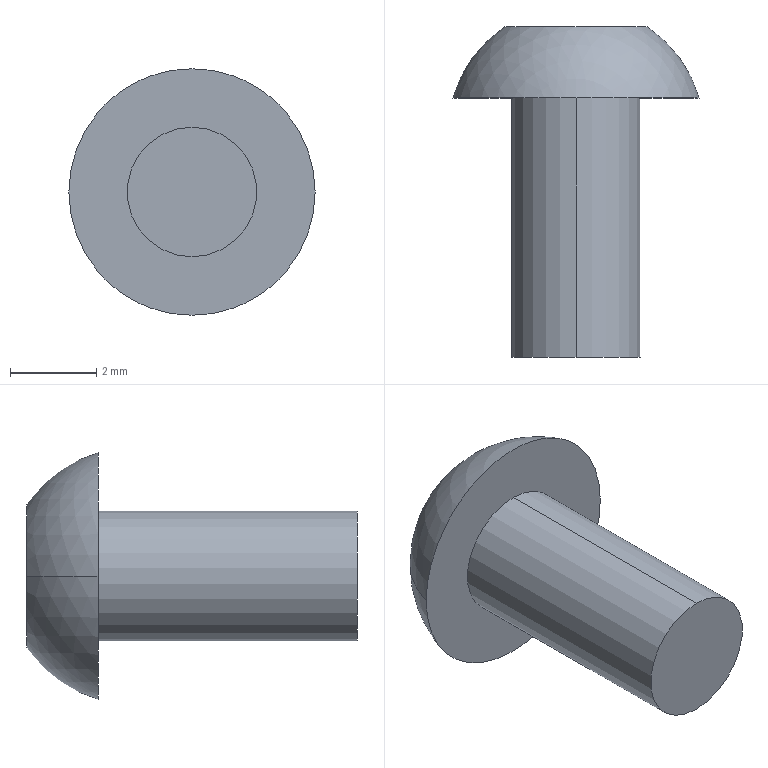Component | SolidWorks | hexagon socket button head screws gb-1 | 1 solid | 19 faces | box 5.7 x 7.65 x 5.7 mm | volume 69 mm3 | plane 15 | sphere 2 | cylinder 2 | commonest cylinder face diameters 3 x2
STEP:
#1=COLOUR_RGB('',0.7922,0.8196,0.9333);
#2=FILL_AREA_STYLE_COLOUR('',#1);
#3=FILL_AREA_STYLE('',(#2));
#4=SURFACE_STYLE_FILL_AREA(#3);
#5=SURFACE_SIDE_STYLE('',(#4));
#6=SURFACE_STYLE_USAGE(.BOTH.,#5);
#7=PRESENTATION_STYLE_ASSIGNMENT((#6));
#8=CARTESIAN_POINT('',(0.7107,0.6105,5.318));
#9=VERTEX_POINT('',#8);
#10=CARTESIAN_POINT('',(0.4863,0.6105,5.318));
#11=VERTEX_POINT('',#10);
#12=CARTESIAN_POINT('',(0.5985,0.6105,5.318));
#13=DIRECTION('',(0.,1.,-0.));
#14=DIRECTION('',(0.,0.,1.));
#15=AXIS2_PLACEMENT_3D('',#12,#13,#14);
#16=CIRCLE('',#15,0.1122);
#17=EDGE_CURVE('',#9,#11,#16,.T.);
#18=ORIENTED_EDGE('',*,*,#17,.T.);
#19=CARTESIAN_POINT('',(0.5336,0.6754,5.318));
#20=VERTEX_POINT('',#19);
#21=CARTESIAN_POINT('',(0.5985,0.5785,5.318));
#22=DIRECTION('',(0.,-0.,-1.));
#23=DIRECTION('',(-1.,0.,0.));
#24=AXIS2_PLACEMENT_3D('',#21,#22,#23);
#25=CIRCLE('',#24,0.1167);
#26=EDGE_CURVE('',#11,#20,#25,.T.);
#27=ORIENTED_EDGE('',*,*,#26,.T.);
#28=CARTESIAN_POINT('',(0.6635,0.6754,5.318));
#29=VERTEX_POINT('',#28);
#30=CARTESIAN_POINT('',(0.5985,0.6754,5.318));
#31=DIRECTION('',(0.,1.,-0.));
#32=DIRECTION('',(0.,0.,1.));
#33=AXIS2_PLACEMENT_3D('',#30,#31,#32);
#34=CIRCLE('',#33,0.06496);
#35=EDGE_CURVE('',#29,#20,#34,.T.);
#36=ORIENTED_EDGE('',*,*,#35,.F.);
#37=CARTESIAN_POINT('',(0.5985,0.5785,5.318));
#38=DIRECTION('',(-0.,0.,1.));
#39=DIRECTION('',(1.,0.,0.));
#40=AXIS2_PLACEMENT_3D('',#37,#38,#39);
#41=CIRCLE('',#40,0.1167);
#42=EDGE_CURVE('',#9,#29,#41,.T.);
#43=ORIENTED_EDGE('',*,*,#42,.F.);
#44=EDGE_LOOP('',(#18,#27,#36,#43));
#45=FACE_OUTER_BOUND('',#44,.T.);
#46=CARTESIAN_POINT('',(0.5985,0.5785,5.318));
#47=DIRECTION('',(0.,-0.,-1.));
#48=DIRECTION('',(1.,0.,0.));
#49=AXIS2_PLACEMENT_3D('',#46,#47,#48);
#50=SPHERICAL_SURFACE('',#49,0.1167);
#51=ADVANCED_FACE('',(#45),#50,.T.);
#52=CARTESIAN_POINT('',(0.5985,0.3743,5.259));
#53=VERTEX_POINT('',#52);
#54=CARTESIAN_POINT('',(0.5985,0.3743,5.377));
#55=VERTEX_POINT('',#54);
#56=CARTESIAN_POINT('',(0.5985,0.3743,5.318));
#57=DIRECTION('',(-0.,-1.,0.));
#58=DIRECTION('',(0.,0.,-1.));
#59=AXIS2_PLACEMENT_3D('',#56,#57,#58);
#60=CIRCLE('',#59,0.05906);
#61=EDGE_CURVE('',#53,#55,#60,.T.);
#62=ORIENTED_EDGE('',*,*,#61,.F.);
#63=CARTESIAN_POINT('',(0.5985,0.6105,5.259));
#64=VERTEX_POINT('',#63);
#65=CARTESIAN_POINT('',(0.5985,0.3743,5.259));
#66=DIRECTION('',(0.,1.,-0.));
#67=VECTOR('',#66,39.37);
#68=LINE('',#65,#67);
#69=EDGE_CURVE('',#53,#64,#68,.T.);
#70=ORIENTED_EDGE('',*,*,#69,.T.);
#71=CARTESIAN_POINT('',(0.5985,0.6105,5.377));
#72=VERTEX_POINT('',#71);
#73=CARTESIAN_POINT('',(0.5985,0.6105,5.318));
#74=DIRECTION('',(-0.,-1.,0.));
#75=DIRECTION('',(0.,0.,-1.));
#76=AXIS2_PLACEMENT_3D('',#73,#74,#75);
#77=CIRCLE('',#76,0.05906);
#78=EDGE_CURVE('',#64,#72,#77,.T.);
#79=ORIENTED_EDGE('',*,*,#78,.T.);
#80=CARTESIAN_POINT('',(0.5985,0.3743,5.377));
#81=DIRECTION('',(0.,1.,-0.));
#82=VECTOR('',#81,39.37);
#83=LINE('',#80,#82);
#84=EDGE_CURVE('',#55,#72,#83,.T.);
#85=ORIENTED_EDGE('',*,*,#84,.F.);
#86=EDGE_LOOP('',(#62,#70,#79,#85));
#87=FACE_OUTER_BOUND('',#86,.T.);
#88=CARTESIAN_POINT('',(0.5985,0.3743,5.318));
#89=DIRECTION('',(0.,1.,-0.));
#90=DIRECTION('',(0.,0.,1.));
#91=AXIS2_PLACEMENT_3D('',#88,#89,#90);
#92=CYLINDRICAL_SURFACE('',#91,0.05906);
#93=ADVANCED_FACE('',(#87),#92,.T.);
#94=ORIENTED_EDGE('',*,*,#35,.T.);
#95=CARTESIAN_POINT('',(0.5985,0.6754,5.318));
#96=DIRECTION('',(0.,1.,-0.));
#97=DIRECTION('',(0.,0.,1.));
#98=AXIS2_PLACEMENT_3D('',#95,#96,#97);
#99=CIRCLE('',#98,0.06496);
#100=EDGE_CURVE('',#20,#29,#99,.T.);
#101=ORIENTED_EDGE('',*,*,#100,.T.);
#102=EDGE_LOOP('',(#94,#101));
#103=FACE_OUTER_BOUND('',#102,.T.);
#104=CARTESIAN_POINT('',(0.5592,0.6754,5.295));
#105=VERTEX_POINT('',#104);
#106=CARTESIAN_POINT('',(0.5985,0.6754,5.272));
#107=VERTEX_POINT('',#106);
#108=CARTESIAN_POINT('',(0.5592,0.6754,5.295));
#109=DIRECTION('',(0.866,-0.,-0.5));
#110=VECTOR('',#109,39.37);
#111=LINE('',#108,#110);
#112=EDGE_CURVE('',#105,#107,#111,.T.);
#113=ORIENTED_EDGE('',*,*,#112,.T.);
#114=CARTESIAN_POINT('',(0.6379,0.6754,5.295));
#115=VERTEX_POINT('',#114);
#116=CARTESIAN_POINT('',(0.5985,0.6754,5.272));
#117=DIRECTION('',(0.866,-0.,0.5));
#118=VECTOR('',#117,39.37);
#119=LINE('',#116,#118);
#120=EDGE_CURVE('',#107,#115,#119,.T.);
#121=ORIENTED_EDGE('',*,*,#120,.T.);
#122=CARTESIAN_POINT('',(0.6379,0.6754,5.34));
#123=VERTEX_POINT('',#122);
#124=CARTESIAN_POINT('',(0.6379,0.6754,5.295));
#125=DIRECTION('',(-0.,0.,1.));
#126=VECTOR('',#125,39.37);
#127=LINE('',#124,#126);
#128=EDGE_CURVE('',#115,#123,#127,.T.);
#129=ORIENTED_EDGE('',*,*,#128,.T.);
#130=CARTESIAN_POINT('',(0.5985,0.6754,5.363));
#131=VERTEX_POINT('',#130);
#132=CARTESIAN_POINT('',(0.6379,0.6754,5.34));
#133=DIRECTION('',(-0.866,0.,0.5));
#134=VECTOR('',#133,39.37);
#135=LINE('',#132,#134);
#136=EDGE_CURVE('',#123,#131,#135,.T.);
#137=ORIENTED_EDGE('',*,*,#136,.T.);
#138=CARTESIAN_POINT('',(0.5592,0.6754,5.34));
#139=VERTEX_POINT('',#138);
#140=CARTESIAN_POINT('',(0.5985,0.6754,5.363));
#141=DIRECTION('',(-0.866,0.,-0.5));
#142=VECTOR('',#141,39.37);
#143=LINE('',#140,#142);
#144=EDGE_CURVE('',#131,#139,#143,.T.);
#145=ORIENTED_EDGE('',*,*,#144,.T.);
#146=CARTESIAN_POINT('',(0.5592,0.6754,5.34));
#147=DIRECTION('',(0.,-0.,-1.));
#148=VECTOR('',#147,39.37);
#149=LINE('',#146,#148);
#150=EDGE_CURVE('',#139,#105,#149,.T.);
#151=ORIENTED_EDGE('',*,*,#150,.T.);
#152=EDGE_LOOP('',(#113,#121,#129,#137,#145,#151));
#153=FACE_BOUND('',#152,.T.);
#154=CARTESIAN_POINT('',(0.5985,0.6754,5.318));
#155=DIRECTION('',(-0.,-1.,0.));
#156=DIRECTION('',(0.,-0.,-1.));
#157=AXIS2_PLACEMENT_3D('',#154,#155,#156);
#158=PLANE('',#157);
#159=ADVANCED_FACE('',(#103,#153),#158,.F.);
#160=ORIENTED_EDGE('',*,*,#17,.F.);
#161=CARTESIAN_POINT('',(0.5985,0.6105,5.318));
#162=DIRECTION('',(0.,1.,-0.));
#163=DIRECTION('',(0.,0.,1.));
#164=AXIS2_PLACEMENT_3D('',#161,#162,#163);
#165=CIRCLE('',#164,0.1122);
#166=EDGE_CURVE('',#11,#9,#165,.T.);
#167=ORIENTED_EDGE('',*,*,#166,.F.);
#168=EDGE_LOOP('',(#160,#167));
#169=FACE_OUTER_BOUND('',#168,.T.);
#170=CARTESIAN_POINT('',(0.5985,0.6105,5.318));
#171=DIRECTION('',(-0.,-1.,0.));
#172=DIRECTION('',(0.,0.,-1.));
#173=AXIS2_PLACEMENT_3D('',#170,#171,#172);
#174=CIRCLE('',#173,0.05906);
#175=EDGE_CURVE('',#72,#64,#174,.T.);
#176=ORIENTED_EDGE('',*,*,#175,.F.);
#177=ORIENTED_EDGE('',*,*,#78,.F.);
#178=EDGE_LOOP('',(#176,#177));
#179=FACE_BOUND('',#178,.T.);
#180=CARTESIAN_POINT('',(0.5985,0.6105,5.318));
#181=DIRECTION('',(-0.,-1.,0.));
#182=DIRECTION('',(0.,-0.,-1.));
#183=AXIS2_PLACEMENT_3D('',#180,#181,#182);
#184=PLANE('',#183);
#185=ADVANCED_FACE('',(#169,#179),#184,.T.);
#186=ORIENTED_EDGE('',*,*,#69,.F.);
#187=CARTESIAN_POINT('',(0.5985,0.3743,5.318));
#188=DIRECTION('',(-0.,-1.,0.));
#189=DIRECTION('',(0.,0.,-1.));
#190=AXIS2_PLACEMENT_3D('',#187,#188,#189);
#191=CIRCLE('',#190,0.05906);
#192=EDGE_CURVE('',#55,#53,#191,.T.);
#193=ORIENTED_EDGE('',*,*,#192,.F.);
#194=ORIENTED_EDGE('',*,*,#84,.T.);
#195=ORIENTED_EDGE('',*,*,#175,.T.);
#196=EDGE_LOOP('',(#186,#193,#194,#195));
#197=FACE_OUTER_BOUND('',#196,.T.);
#198=CARTESIAN_POINT('',(0.5985,0.3743,5.318));
#199=DIRECTION('',(0.,1.,-0.));
#200=DIRECTION('',(0.,0.,1.));
#201=AXIS2_PLACEMENT_3D('',#198,#199,#200);
#202=CYLINDRICAL_SURFACE('',#201,0.05906);
#203=ADVANCED_FACE('',(#197),#202,.T.);
#204=ORIENTED_EDGE('',*,*,#192,.T.);
#205=ORIENTED_EDGE('',*,*,#61,.T.);
#206=EDGE_LOOP('',(#204,#205));
#207=FACE_OUTER_BOUND('',#206,.T.);
#208=CARTESIAN_POINT('',(0.5985,0.3743,5.318));
#209=DIRECTION('',(-0.,-1.,0.));
#210=DIRECTION('',(0.,-0.,-1.));
#211=AXIS2_PLACEMENT_3D('',#208,#209,#210);
#212=PLANE('',#211);
#213=ADVANCED_FACE('',(#207),#212,.T.);
#214=ORIENTED_EDGE('',*,*,#26,.F.);
#215=ORIENTED_EDGE('',*,*,#166,.T.);
#216=ORIENTED_EDGE('',*,*,#42,.T.);
#217=ORIENTED_EDGE('',*,*,#100,.F.);
#218=EDGE_LOOP('',(#214,#215,#216,#217));
#219=FACE_OUTER_BOUND('',#218,.T.);
#220=CARTESIAN_POINT('',(0.5985,0.5785,5.318));
#221=DIRECTION('',(0.,-0.,-1.));
#222=DIRECTION('',(1.,0.,0.));
#223=AXIS2_PLACEMENT_3D('',#220,#221,#222);
#224=SPHERICAL_SURFACE('',#223,0.1167);
#225=ADVANCED_FACE('',(#219),#224,.T.);
#226=ORIENTED_EDGE('',*,*,#112,.F.);
#227=CARTESIAN_POINT('',(0.5592,0.6345,5.295));
#228=VERTEX_POINT('',#227);
#229=CARTESIAN_POINT('',(0.5592,0.6345,5.295));
#230=DIRECTION('',(0.,1.,-0.));
#231=VECTOR('',#230,39.37);
#232=LINE('',#229,#231);
#233=EDGE_CURVE('',#228,#105,#232,.T.);
#234=ORIENTED_EDGE('',*,*,#233,.F.);
#235=CARTESIAN_POINT('',(0.5985,0.6345,5.272));
#236=VERTEX_POINT('',#235);
#237=CARTESIAN_POINT('',(0.5592,0.6345,5.295));
#238=DIRECTION('',(0.866,-0.,-0.5));
#239=VECTOR('',#238,39.37);
#240=LINE('',#237,#239);
#241=EDGE_CURVE('',#228,#236,#240,.T.);
#242=ORIENTED_EDGE('',*,*,#241,.T.);
#243=CARTESIAN_POINT('',(0.5985,0.6345,5.272));
#244=DIRECTION('',(0.,1.,-0.));
#245=VECTOR('',#244,39.37);
#246=LINE('',#243,#245);
#247=EDGE_CURVE('',#236,#107,#246,.T.);
#248=ORIENTED_EDGE('',*,*,#247,.T.);
#249=EDGE_LOOP('',(#226,#234,#242,#248));
#250=FACE_OUTER_BOUND('',#249,.T.);
#251=CARTESIAN_POINT('',(0.5592,0.6345,5.295));
#252=DIRECTION('',(0.5,0.,0.866));
#253=DIRECTION('',(-0.866,0.,0.5));
#254=AXIS2_PLACEMENT_3D('',#251,#252,#253);
#255=PLANE('',#254);
#256=ADVANCED_FACE('',(#250),#255,.T.);
#257=ORIENTED_EDGE('',*,*,#120,.F.);
#258=ORIENTED_EDGE('',*,*,#247,.F.);
#259=CARTESIAN_POINT('',(0.6379,0.6345,5.295));
#260=VERTEX_POINT('',#259);
#261=CARTESIAN_POINT('',(0.5985,0.6345,5.272));
#262=DIRECTION('',(0.866,-0.,0.5));
#263=VECTOR('',#262,39.37);
#264=LINE('',#261,#263);
#265=EDGE_CURVE('',#236,#260,#264,.T.);
#266=ORIENTED_EDGE('',*,*,#265,.T.);
#267=CARTESIAN_POINT('',(0.6379,0.6345,5.295));
#268=DIRECTION('',(0.,1.,-0.));
#269=VECTOR('',#268,39.37);
#270=LINE('',#267,#269);
#271=EDGE_CURVE('',#260,#115,#270,.T.);
#272=ORIENTED_EDGE('',*,*,#271,.T.);
#273=EDGE_LOOP('',(#257,#258,#266,#272));
#274=FACE_OUTER_BOUND('',#273,.T.);
#275=CARTESIAN_POINT('',(0.5985,0.6345,5.272));
#276=DIRECTION('',(-0.5,0.,0.866));
#277=DIRECTION('',(-0.866,0.,-0.5));
#278=AXIS2_PLACEMENT_3D('',#275,#276,#277);
#279=PLANE('',#278);
#280=ADVANCED_FACE('',(#274),#279,.T.);
#281=ORIENTED_EDGE('',*,*,#128,.F.);
#282=ORIENTED_EDGE('',*,*,#271,.F.);
#283=CARTESIAN_POINT('',(0.6379,0.6345,5.34));
#284=VERTEX_POINT('',#283);
#285=CARTESIAN_POINT('',(0.6379,0.6345,5.295));
#286=DIRECTION('',(-0.,0.,1.));
#287=VECTOR('',#286,39.37);
#288=LINE('',#285,#287);
#289=EDGE_CURVE('',#260,#284,#288,.T.);
#290=ORIENTED_EDGE('',*,*,#289,.T.);
#291=CARTESIAN_POINT('',(0.6379,0.6345,5.34));
#292=DIRECTION('',(0.,1.,-0.));
#293=VECTOR('',#292,39.37);
#294=LINE('',#291,#293);
#295=EDGE_CURVE('',#284,#123,#294,.T.);
#296=ORIENTED_EDGE('',*,*,#295,.T.);
#297=EDGE_LOOP('',(#281,#282,#290,#296));
#298=FACE_OUTER_BOUND('',#297,.T.);
#299=CARTESIAN_POINT('',(0.6379,0.6345,5.295));
#300=DIRECTION('',(-1.,0.,-0.));
#301=DIRECTION('',(0.,-0.,-1.));
#302=AXIS2_PLACEMENT_3D('',#299,#300,#301);
#303=PLANE('',#302);
#304=ADVANCED_FACE('',(#298),#303,.T.);
#305=ORIENTED_EDGE('',*,*,#136,.F.);
#306=ORIENTED_EDGE('',*,*,#295,.F.);
#307=CARTESIAN_POINT('',(0.5985,0.6345,5.363));
#308=VERTEX_POINT('',#307);
#309=CARTESIAN_POINT('',(0.6379,0.6345,5.34));
#310=DIRECTION('',(-0.866,0.,0.5));
#311=VECTOR('',#310,39.37);
#312=LINE('',#309,#311);
#313=EDGE_CURVE('',#284,#308,#312,.T.);
#314=ORIENTED_EDGE('',*,*,#313,.T.);
#315=CARTESIAN_POINT('',(0.5985,0.6345,5.363));
#316=DIRECTION('',(0.,1.,-0.));
#317=VECTOR('',#316,39.37);
#318=LINE('',#315,#317);
#319=EDGE_CURVE('',#308,#131,#318,.T.);
#320=ORIENTED_EDGE('',*,*,#319,.T.);
#321=EDGE_LOOP('',(#305,#306,#314,#320));
#322=FACE_OUTER_BOUND('',#321,.T.);
#323=CARTESIAN_POINT('',(0.6379,0.6345,5.34));
#324=DIRECTION('',(-0.5,-0.,-0.866));
#325=DIRECTION('',(0.866,-0.,-0.5));
#326=AXIS2_PLACEMENT_3D('',#323,#324,#325);
#327=PLANE('',#326);
#328=ADVANCED_FACE('',(#322),#327,.T.);
#329=ORIENTED_EDGE('',*,*,#144,.F.);
#330=ORIENTED_EDGE('',*,*,#319,.F.);
#331=CARTESIAN_POINT('',(0.5592,0.6345,5.34));
#332=VERTEX_POINT('',#331);
#333=CARTESIAN_POINT('',(0.5985,0.6345,5.363));
#334=DIRECTION('',(-0.866,0.,-0.5));
#335=VECTOR('',#334,39.37);
#336=LINE('',#333,#335);
#337=EDGE_CURVE('',#308,#332,#336,.T.);
#338=ORIENTED_EDGE('',*,*,#337,.T.);
#339=CARTESIAN_POINT('',(0.5592,0.6345,5.34));
#340=DIRECTION('',(0.,1.,-0.));
#341=VECTOR('',#340,39.37);
#342=LINE('',#339,#341);
#343=EDGE_CURVE('',#332,#139,#342,.T.);
#344=ORIENTED_EDGE('',*,*,#343,.T.);
#345=EDGE_LOOP('',(#329,#330,#338,#344));
#346=FACE_OUTER_BOUND('',#345,.T.);
#347=CARTESIAN_POINT('',(0.5985,0.6345,5.363));
#348=DIRECTION('',(0.5,-0.,-0.866));
#349=DIRECTION('',(0.866,-0.,0.5));
#350=AXIS2_PLACEMENT_3D('',#347,#348,#349);
#351=PLANE('',#350);
#352=ADVANCED_FACE('',(#346),#351,.T.);
#353=ORIENTED_EDGE('',*,*,#150,.F.);
#354=ORIENTED_EDGE('',*,*,#343,.F.);
#355=CARTESIAN_POINT('',(0.5592,0.6345,5.34));
#356=DIRECTION('',(0.,-0.,-1.));
#357=VECTOR('',#356,39.37);
#358=LINE('',#355,#357);
#359=EDGE_CURVE('',#332,#228,#358,.T.);
#360=ORIENTED_EDGE('',*,*,#359,.T.);
#361=ORIENTED_EDGE('',*,*,#233,.T.);
#362=EDGE_LOOP('',(#353,#354,#360,#361));
#363=FACE_OUTER_BOUND('',#362,.T.);
#364=CARTESIAN_POINT('',(0.5592,0.6345,5.34));
#365=DIRECTION('',(1.,-0.,0.));
#366=DIRECTION('',(-0.,0.,1.));
#367=AXIS2_PLACEMENT_3D('',#364,#365,#366);
#368=PLANE('',#367);
#369=ADVANCED_FACE('',(#363),#368,.T.);
#370=ORIENTED_EDGE('',*,*,#337,.F.);
#371=CARTESIAN_POINT('',(0.5985,0.6118,5.318));
#372=VERTEX_POINT('',#371);
#373=CARTESIAN_POINT('',(0.5985,0.6345,5.363));
#374=DIRECTION('',(-0.,0.4472,0.8944));
#375=VECTOR('',#374,39.37);
#376=LINE('',#373,#375);
#377=EDGE_CURVE('',#372,#308,#376,.T.);
#378=ORIENTED_EDGE('',*,*,#377,.F.);
#379=CARTESIAN_POINT('',(0.5592,0.6345,5.34));
#380=DIRECTION('',(-0.7746,0.4472,0.4472));
#381=VECTOR('',#380,39.37);
#382=LINE('',#379,#381);
#383=EDGE_CURVE('',#372,#332,#382,.T.);
#384=ORIENTED_EDGE('',*,*,#383,.T.);
#385=EDGE_LOOP('',(#370,#378,#384));
#386=FACE_OUTER_BOUND('',#385,.T.);
#387=CARTESIAN_POINT('',(0.5985,0.6345,5.363));
#388=DIRECTION('',(-0.25,-0.866,0.433));
#389=DIRECTION('',(0.,-0.4472,-0.8944));
#390=AXIS2_PLACEMENT_3D('',#387,#388,#389);
#391=PLANE('',#390);
#392=ADVANCED_FACE('',(#386),#391,.F.);
#393=ORIENTED_EDGE('',*,*,#359,.F.);
#394=ORIENTED_EDGE('',*,*,#383,.F.);
#395=CARTESIAN_POINT('',(0.5592,0.6345,5.295));
#396=DIRECTION('',(-0.7746,0.4472,-0.4472));
#397=VECTOR('',#396,39.37);
#398=LINE('',#395,#397);
#399=EDGE_CURVE('',#372,#228,#398,.T.);
#400=ORIENTED_EDGE('',*,*,#399,.T.);
#401=EDGE_LOOP('',(#393,#394,#400));
#402=FACE_OUTER_BOUND('',#401,.T.);
#403=CARTESIAN_POINT('',(0.5592,0.6345,5.34));
#404=DIRECTION('',(-0.5,-0.866,0.));
#405=DIRECTION('',(0.866,-0.5,0.));
#406=AXIS2_PLACEMENT_3D('',#403,#404,#405);
#407=PLANE('',#406);
#408=ADVANCED_FACE('',(#402),#407,.F.);
#409=ORIENTED_EDGE('',*,*,#241,.F.);
#410=ORIENTED_EDGE('',*,*,#399,.F.);
#411=CARTESIAN_POINT('',(0.5985,0.6345,5.272));
#412=DIRECTION('',(0.,0.4472,-0.8944));
#413=VECTOR('',#412,39.37);
#414=LINE('',#411,#413);
#415=EDGE_CURVE('',#372,#236,#414,.T.);
#416=ORIENTED_EDGE('',*,*,#415,.T.);
#417=EDGE_LOOP('',(#409,#410,#416));
#418=FACE_OUTER_BOUND('',#417,.T.);
#419=CARTESIAN_POINT('',(0.5592,0.6345,5.295));
#420=DIRECTION('',(-0.25,-0.866,-0.433));
#421=DIRECTION('',(0.,0.4472,-0.8944));
#422=AXIS2_PLACEMENT_3D('',#419,#420,#421);
#423=PLANE('',#422);
#424=ADVANCED_FACE('',(#418),#423,.F.);
#425=ORIENTED_EDGE('',*,*,#265,.F.);
#426=ORIENTED_EDGE('',*,*,#415,.F.);
#427=CARTESIAN_POINT('',(0.6379,0.6345,5.295));
#428=DIRECTION('',(0.7746,0.4472,-0.4472));
#429=VECTOR('',#428,39.37);
#430=LINE('',#427,#429);
#431=EDGE_CURVE('',#372,#260,#430,.T.);
#432=ORIENTED_EDGE('',*,*,#431,.T.);
#433=EDGE_LOOP('',(#425,#426,#432));
#434=FACE_OUTER_BOUND('',#433,.T.);
#435=CARTESIAN_POINT('',(0.5985,0.6345,5.272));
#436=DIRECTION('',(0.25,-0.866,-0.433));
#437=DIRECTION('',(0.,0.4472,-0.8944));
#438=AXIS2_PLACEMENT_3D('',#435,#436,#437);
#439=PLANE('',#438);
#440=ADVANCED_FACE('',(#434),#439,.F.);
#441=ORIENTED_EDGE('',*,*,#289,.F.);
#442=ORIENTED_EDGE('',*,*,#431,.F.);
#443=CARTESIAN_POINT('',(0.6379,0.6345,5.34));
#444=DIRECTION('',(0.7746,0.4472,0.4472));
#445=VECTOR('',#444,39.37);
#446=LINE('',#443,#445);
#447=EDGE_CURVE('',#372,#284,#446,.T.);
#448=ORIENTED_EDGE('',*,*,#447,.T.);
#449=EDGE_LOOP('',(#441,#442,#448));
#450=FACE_OUTER_BOUND('',#449,.T.);
#451=CARTESIAN_POINT('',(0.6379,0.6345,5.295));
#452=DIRECTION('',(0.5,-0.866,0.));
#453=DIRECTION('',(0.866,0.5,0.));
#454=AXIS2_PLACEMENT_3D('',#451,#452,#453);
#455=PLANE('',#454);
#456=ADVANCED_FACE('',(#450),#455,.F.);
#457=ORIENTED_EDGE('',*,*,#313,.F.);
#458=ORIENTED_EDGE('',*,*,#447,.F.);
#459=ORIENTED_EDGE('',*,*,#377,.T.);
#460=EDGE_LOOP('',(#457,#458,#459));
#461=FACE_OUTER_BOUND('',#460,.T.);
#462=CARTESIAN_POINT('',(0.6379,0.6345,5.34));
#463=DIRECTION('',(0.25,-0.866,0.433));
#464=DIRECTION('',(0.,-0.4472,-0.8944));
#465=AXIS2_PLACEMENT_3D('',#462,#463,#464);
#466=PLANE('',#465);
#467=ADVANCED_FACE('',(#461),#466,.F.);
#468=CLOSED_SHELL('',(#51,#93,#159,#185,#203,#213,#225,#256,#280,#304,#328,#352,#369,#392,#408,#424,#440,#456,#467));
#469=MANIFOLD_SOLID_BREP('',#468);
#470=STYLED_ITEM('',(#7),#469);
#471=(LENGTH_UNIT()NAMED_UNIT(*)SI_UNIT($,.METRE.));
#472=LENGTH_MEASURE_WITH_UNIT(LENGTH_MEASURE(0.0254),#471);
#473=DIMENSIONAL_EXPONENTS(1.,0.,0.,0.,0.,0.,0.);
#474=(CONVERSION_BASED_UNIT('',#472)LENGTH_UNIT()NAMED_UNIT(#473));
#475=UNCERTAINTY_MEASURE_WITH_UNIT(LENGTH_MEASURE(0.00001),#474,'','');
#476=(NAMED_UNIT(*)PLANE_ANGLE_UNIT()SI_UNIT($,.RADIAN.));
#477=(NAMED_UNIT(*)SI_UNIT($,.STERADIAN.)SOLID_ANGLE_UNIT());
#478=(GEOMETRIC_REPRESENTATION_CONTEXT(3)GLOBAL_UNCERTAINTY_ASSIGNED_CONTEXT((#475))GLOBAL_UNIT_ASSIGNED_CONTEXT((#474,#476,#477))REPRESENTATION_CONTEXT('',''));
#479=MECHANICAL_DESIGN_GEOMETRIC_PRESENTATION_REPRESENTATION('',(#470),#478);
#480=PRESENTATION_LAYER_ASSIGNMENT('','',(#470));
#481=CARTESIAN_POINT('',(0.,0.,0.));
#482=DIRECTION('',(0.,0.,1.));
#483=DIRECTION('',(1.,0.,0.));
#484=AXIS2_PLACEMENT_3D('',#481,#482,#483);
#485=(LENGTH_UNIT()NAMED_UNIT(*)SI_UNIT($,.METRE.));
#486=LENGTH_MEASURE_WITH_UNIT(LENGTH_MEASURE(0.0254),#485);
#487=DIMENSIONAL_EXPONENTS(1.,0.,0.,0.,0.,0.,0.);
#488=(CONVERSION_BASED_UNIT('',#486)LENGTH_UNIT()NAMED_UNIT(#487));
#489=UNCERTAINTY_MEASURE_WITH_UNIT(LENGTH_MEASURE(0.00001),#488,'','');
#490=(NAMED_UNIT(*)PLANE_ANGLE_UNIT()SI_UNIT($,.RADIAN.));
#491=(NAMED_UNIT(*)SI_UNIT($,.STERADIAN.)SOLID_ANGLE_UNIT());
#492=(GEOMETRIC_REPRESENTATION_CONTEXT(3)GLOBAL_UNCERTAINTY_ASSIGNED_CONTEXT((#489))GLOBAL_UNIT_ASSIGNED_CONTEXT((#488,#490,#491))REPRESENTATION_CONTEXT('',''));
#493=ADVANCED_BREP_SHAPE_REPRESENTATION('',(#469,#484),#492);